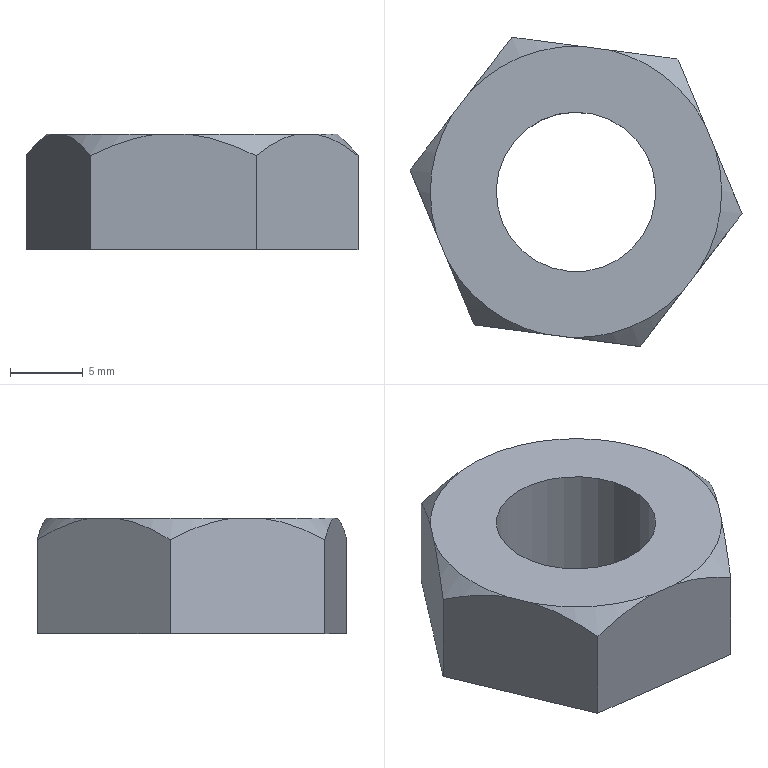Component | NX | HEXNUTM12 | 1 solid | 15 faces | volume 1997 mm3 | plane 8 | cone 6 | cylinder 1 | commonest cylinder face diameters 11 x1